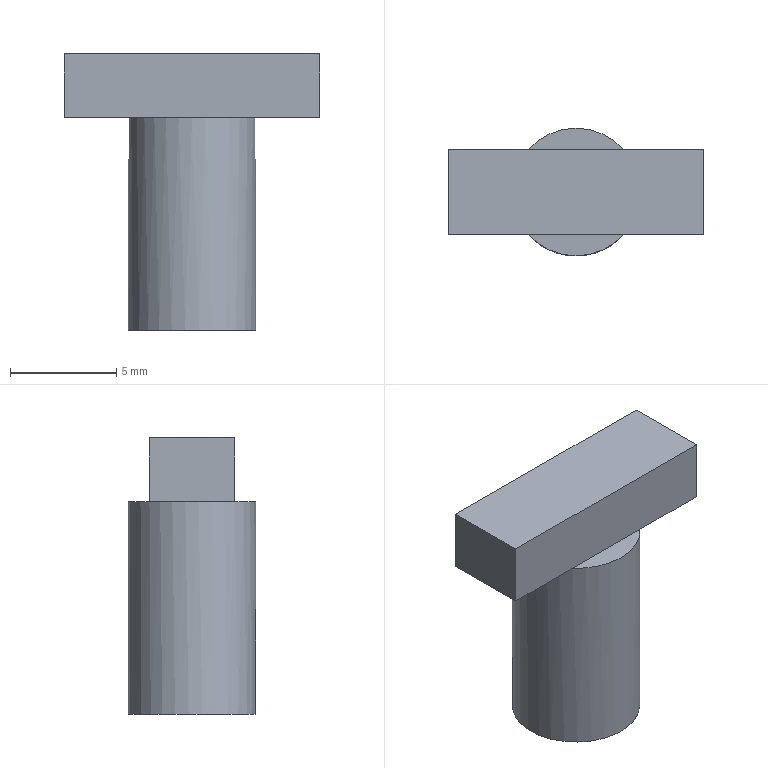Component | NX | DETENT_PIN | 1 solid | 11 faces | box 12 x 6 x 13 mm | volume 427 mm3 | plane 10 | cylinder 1 | commonest cylinder face diameters 6 x1
STEP:
#1=CARTESIAN_POINT('',(0.,0.,0.));
#2=DIRECTION('',(0.,0.,1.));
#3=DIRECTION('',(1.,0.,0.));
#4=AXIS2_PLACEMENT_3D('',#1,#2,#3);
#5=CARTESIAN_POINT('',(12.764,-2.,126.));
#6=VERTEX_POINT('',#5);
#7=CARTESIAN_POINT('',(17.236,-2.,126.));
#8=VERTEX_POINT('',#7);
#9=CARTESIAN_POINT('',(9.,-2.,126.));
#10=DIRECTION('',(1.,0.,0.));
#11=VECTOR('',#10,1.);
#12=LINE('',#9,#11);
#13=CARTESIAN_POINT('',(15.,0.,126.));
#14=DIRECTION('',(0.,0.,1.));
#15=DIRECTION('',(0.,1.,0.));
#16=AXIS2_PLACEMENT_3D('',#13,#14,#15);
#17=PLANE('',#16);
#18=CARTESIAN_POINT('',(-2.,6.));
#19=DIRECTION('',(0.,-1.));
#20=VECTOR('',#19,1.);
#21=LINE('',#18,#20);
#22=(GEOMETRIC_REPRESENTATION_CONTEXT(2)PARAMETRIC_REPRESENTATION_CONTEXT()REPRESENTATION_CONTEXT('',''));
#23=DEFINITIONAL_REPRESENTATION('',(#21),#22);
#24=PCURVE('',#17,#23);
#25=CARTESIAN_POINT('',(9.,-2.,129.));
#26=DIRECTION('',(0.,1.,0.));
#27=DIRECTION('',(0.,0.,-1.));
#28=AXIS2_PLACEMENT_3D('',#25,#26,#27);
#29=PLANE('',#28);
#30=CARTESIAN_POINT('',(3.,0.));
#31=DIRECTION('',(0.,-1.));
#32=VECTOR('',#31,1.);
#33=LINE('',#30,#32);
#34=(GEOMETRIC_REPRESENTATION_CONTEXT(2)PARAMETRIC_REPRESENTATION_CONTEXT()REPRESENTATION_CONTEXT('',''));
#35=DEFINITIONAL_REPRESENTATION('',(#33),#34);
#36=PCURVE('',#29,#35);
#37=SURFACE_CURVE('',#12,(#24,#36),.PCURVE_S1.);
#38=EDGE_CURVE('',#6,#8,#37,.T.);
#39=ORIENTED_EDGE('',*,*,#38,.F.);
#40=CARTESIAN_POINT('',(15.,0.,126.));
#41=DIRECTION('',(0.,0.,-1.));
#42=DIRECTION('',(0.,1.,0.));
#43=AXIS2_PLACEMENT_3D('',#40,#41,#42);
#44=CIRCLE('',#43,3.);
#45=CARTESIAN_POINT('',(3.,0.));
#46=CARTESIAN_POINT('',(3.,-5.196));
#47=CARTESIAN_POINT('',(-1.5,-2.598));
#48=CARTESIAN_POINT('',(-6.,-0.));
#49=CARTESIAN_POINT('',(-1.5,2.598));
#50=CARTESIAN_POINT('',(3.,5.196));
#51=CARTESIAN_POINT('',(3.,0.));
#52=(BOUNDED_CURVE()B_SPLINE_CURVE(2,(#45,#46,#47,#48,#49,#50,#51),.UNSPECIFIED.,.T.,.F.)B_SPLINE_CURVE_WITH_KNOTS((1,2,2,2,2,1),(-2.094,0.,2.094,4.189,6.283,8.378),.UNSPECIFIED.)CURVE()GEOMETRIC_REPRESENTATION_ITEM()RATIONAL_B_SPLINE_CURVE((1.,0.5,1.,0.5,1.,0.5,1.))REPRESENTATION_ITEM(''));
#53=(GEOMETRIC_REPRESENTATION_CONTEXT(2)PARAMETRIC_REPRESENTATION_CONTEXT()REPRESENTATION_CONTEXT('',''));
#54=DEFINITIONAL_REPRESENTATION('',(#52),#53);
#55=PCURVE('',#17,#54);
#56=CARTESIAN_POINT('',(15.,0.,126.));
#57=DIRECTION('',(0.,0.,-1.));
#58=DIRECTION('',(0.,1.,0.));
#59=AXIS2_PLACEMENT_3D('',#56,#57,#58);
#60=CYLINDRICAL_SURFACE('',#59,3.);
#61=CARTESIAN_POINT('',(0.,0.));
#62=DIRECTION('',(1.,0.));
#63=VECTOR('',#62,1.);
#64=LINE('',#61,#63);
#65=(GEOMETRIC_REPRESENTATION_CONTEXT(2)PARAMETRIC_REPRESENTATION_CONTEXT()REPRESENTATION_CONTEXT('',''));
#66=DEFINITIONAL_REPRESENTATION('',(#64),#65);
#67=PCURVE('',#60,#66);
#68=SURFACE_CURVE('',#44,(#55,#67),.PCURVE_S1.);
#69=EDGE_CURVE('',#8,#6,#68,.T.);
#70=ORIENTED_EDGE('',*,*,#69,.F.);
#71=EDGE_LOOP('',(#39,#70));
#72=FACE_BOUND('',#71,.T.);
#73=ADVANCED_FACE('',(#72),#17,.T.);
#74=CARTESIAN_POINT('',(15.,3.,116.));
#75=VERTEX_POINT('',#74);
#76=CARTESIAN_POINT('',(15.,0.,116.));
#77=DIRECTION('',(0.,0.,1.));
#78=DIRECTION('',(0.,1.,0.));
#79=AXIS2_PLACEMENT_3D('',#76,#77,#78);
#80=CIRCLE('',#79,3.);
#81=CARTESIAN_POINT('',(15.,0.,116.));
#82=DIRECTION('',(0.,0.,-1.));
#83=DIRECTION('',(0.,-1.,0.));
#84=AXIS2_PLACEMENT_3D('',#81,#82,#83);
#85=PLANE('',#84);
#86=CARTESIAN_POINT('',(-3.,0.));
#87=CARTESIAN_POINT('',(-3.,5.196));
#88=CARTESIAN_POINT('',(1.5,2.598));
#89=CARTESIAN_POINT('',(6.,0.));
#90=CARTESIAN_POINT('',(1.5,-2.598));
#91=CARTESIAN_POINT('',(-3.,-5.196));
#92=CARTESIAN_POINT('',(-3.,0.));
#93=(BOUNDED_CURVE()B_SPLINE_CURVE(2,(#86,#87,#88,#89,#90,#91,#92),.UNSPECIFIED.,.T.,.F.)B_SPLINE_CURVE_WITH_KNOTS((1,2,2,2,2,1),(-2.094,0.,2.094,4.189,6.283,8.378),.UNSPECIFIED.)CURVE()GEOMETRIC_REPRESENTATION_ITEM()RATIONAL_B_SPLINE_CURVE((1.,0.5,1.,0.5,1.,0.5,1.))REPRESENTATION_ITEM(''));
#94=(GEOMETRIC_REPRESENTATION_CONTEXT(2)PARAMETRIC_REPRESENTATION_CONTEXT()REPRESENTATION_CONTEXT('',''));
#95=DEFINITIONAL_REPRESENTATION('',(#93),#94);
#96=PCURVE('',#85,#95);
#97=CARTESIAN_POINT('',(6.283,10.));
#98=DIRECTION('',(-1.,0.));
#99=VECTOR('',#98,1.);
#100=LINE('',#97,#99);
#101=(GEOMETRIC_REPRESENTATION_CONTEXT(2)PARAMETRIC_REPRESENTATION_CONTEXT()REPRESENTATION_CONTEXT('',''));
#102=DEFINITIONAL_REPRESENTATION('',(#100),#101);
#103=PCURVE('',#60,#102);
#104=SURFACE_CURVE('',#80,(#96,#103),.PCURVE_S1.);
#105=EDGE_CURVE('',#75,#75,#104,.T.);
#106=ORIENTED_EDGE('',*,*,#105,.F.);
#107=EDGE_LOOP('',(#106));
#108=FACE_BOUND('',#107,.T.);
#109=ADVANCED_FACE('',(#108),#85,.T.);
#110=CARTESIAN_POINT('',(17.236,2.,126.));
#111=VERTEX_POINT('',#110);
#112=CARTESIAN_POINT('',(12.764,2.,126.));
#113=VERTEX_POINT('',#112);
#114=CARTESIAN_POINT('',(21.,2.,126.));
#115=DIRECTION('',(-1.,0.,0.));
#116=VECTOR('',#115,1.);
#117=LINE('',#114,#116);
#118=CARTESIAN_POINT('',(15.,0.,126.));
#119=DIRECTION('',(0.,0.,1.));
#120=DIRECTION('',(0.,1.,0.));
#121=AXIS2_PLACEMENT_3D('',#118,#119,#120);
#122=PLANE('',#121);
#123=CARTESIAN_POINT('',(2.,-6.));
#124=DIRECTION('',(0.,1.));
#125=VECTOR('',#124,1.);
#126=LINE('',#123,#125);
#127=(GEOMETRIC_REPRESENTATION_CONTEXT(2)PARAMETRIC_REPRESENTATION_CONTEXT()REPRESENTATION_CONTEXT('',''));
#128=DEFINITIONAL_REPRESENTATION('',(#126),#127);
#129=PCURVE('',#122,#128);
#130=CARTESIAN_POINT('',(21.,2.,129.));
#131=DIRECTION('',(0.,-1.,0.));
#132=DIRECTION('',(0.,0.,1.));
#133=AXIS2_PLACEMENT_3D('',#130,#131,#132);
#134=PLANE('',#133);
#135=CARTESIAN_POINT('',(-3.,0.));
#136=DIRECTION('',(0.,1.));
#137=VECTOR('',#136,1.);
#138=LINE('',#135,#137);
#139=(GEOMETRIC_REPRESENTATION_CONTEXT(2)PARAMETRIC_REPRESENTATION_CONTEXT()REPRESENTATION_CONTEXT('',''));
#140=DEFINITIONAL_REPRESENTATION('',(#138),#139);
#141=PCURVE('',#134,#140);
#142=SURFACE_CURVE('',#117,(#129,#141),.PCURVE_S1.);
#143=EDGE_CURVE('',#111,#113,#142,.T.);
#144=ORIENTED_EDGE('',*,*,#143,.F.);
#145=CARTESIAN_POINT('',(15.,3.,126.));
#146=VERTEX_POINT('',#145);
#147=CARTESIAN_POINT('',(15.,0.,126.));
#148=DIRECTION('',(0.,0.,-1.));
#149=DIRECTION('',(0.,1.,0.));
#150=AXIS2_PLACEMENT_3D('',#147,#148,#149);
#151=CIRCLE('',#150,3.);
#152=CARTESIAN_POINT('',(3.,0.));
#153=CARTESIAN_POINT('',(3.,-5.196));
#154=CARTESIAN_POINT('',(-1.5,-2.598));
#155=CARTESIAN_POINT('',(-6.,-0.));
#156=CARTESIAN_POINT('',(-1.5,2.598));
#157=CARTESIAN_POINT('',(3.,5.196));
#158=CARTESIAN_POINT('',(3.,0.));
#159=(BOUNDED_CURVE()B_SPLINE_CURVE(2,(#152,#153,#154,#155,#156,#157,#158),.UNSPECIFIED.,.T.,.F.)B_SPLINE_CURVE_WITH_KNOTS((1,2,2,2,2,1),(-2.094,0.,2.094,4.189,6.283,8.378),.UNSPECIFIED.)CURVE()GEOMETRIC_REPRESENTATION_ITEM()RATIONAL_B_SPLINE_CURVE((1.,0.5,1.,0.5,1.,0.5,1.))REPRESENTATION_ITEM(''));
#160=(GEOMETRIC_REPRESENTATION_CONTEXT(2)PARAMETRIC_REPRESENTATION_CONTEXT()REPRESENTATION_CONTEXT('',''));
#161=DEFINITIONAL_REPRESENTATION('',(#159),#160);
#162=PCURVE('',#122,#161);
#163=CARTESIAN_POINT('',(-6.283,0.));
#164=DIRECTION('',(1.,0.));
#165=VECTOR('',#164,1.);
#166=LINE('',#163,#165);
#167=(GEOMETRIC_REPRESENTATION_CONTEXT(2)PARAMETRIC_REPRESENTATION_CONTEXT()REPRESENTATION_CONTEXT('',''));
#168=DEFINITIONAL_REPRESENTATION('',(#166),#167);
#169=PCURVE('',#60,#168);
#170=SURFACE_CURVE('',#151,(#162,#169),.PCURVE_S1.);
#171=EDGE_CURVE('',#146,#111,#170,.T.);
#172=ORIENTED_EDGE('',*,*,#171,.F.);
#173=CARTESIAN_POINT('',(15.,0.,126.));
#174=DIRECTION('',(0.,0.,-1.));
#175=DIRECTION('',(0.,1.,0.));
#176=AXIS2_PLACEMENT_3D('',#173,#174,#175);
#177=CIRCLE('',#176,3.);
#178=CARTESIAN_POINT('',(3.,0.));
#179=CARTESIAN_POINT('',(3.,-5.196));
#180=CARTESIAN_POINT('',(-1.5,-2.598));
#181=CARTESIAN_POINT('',(-6.,-0.));
#182=CARTESIAN_POINT('',(-1.5,2.598));
#183=CARTESIAN_POINT('',(3.,5.196));
#184=CARTESIAN_POINT('',(3.,0.));
#185=(BOUNDED_CURVE()B_SPLINE_CURVE(2,(#178,#179,#180,#181,#182,#183,#184),.UNSPECIFIED.,.T.,.F.)B_SPLINE_CURVE_WITH_KNOTS((1,2,2,2,2,1),(-2.094,0.,2.094,4.189,6.283,8.378),.UNSPECIFIED.)CURVE()GEOMETRIC_REPRESENTATION_ITEM()RATIONAL_B_SPLINE_CURVE((1.,0.5,1.,0.5,1.,0.5,1.))REPRESENTATION_ITEM(''));
#186=(GEOMETRIC_REPRESENTATION_CONTEXT(2)PARAMETRIC_REPRESENTATION_CONTEXT()REPRESENTATION_CONTEXT('',''));
#187=DEFINITIONAL_REPRESENTATION('',(#185),#186);
#188=PCURVE('',#122,#187);
#189=CARTESIAN_POINT('',(0.,0.));
#190=DIRECTION('',(1.,0.));
#191=VECTOR('',#190,1.);
#192=LINE('',#189,#191);
#193=(GEOMETRIC_REPRESENTATION_CONTEXT(2)PARAMETRIC_REPRESENTATION_CONTEXT()REPRESENTATION_CONTEXT('',''));
#194=DEFINITIONAL_REPRESENTATION('',(#192),#193);
#195=PCURVE('',#60,#194);
#196=SURFACE_CURVE('',#177,(#188,#195),.PCURVE_S1.);
#197=EDGE_CURVE('',#113,#146,#196,.T.);
#198=ORIENTED_EDGE('',*,*,#197,.F.);
#199=EDGE_LOOP('',(#144,#172,#198));
#200=FACE_BOUND('',#199,.T.);
#201=ADVANCED_FACE('',(#200),#122,.T.);
#202=ORIENTED_EDGE('',*,*,#105,.T.);
#203=CARTESIAN_POINT('',(15.,3.,126.));
#204=CARTESIAN_POINT('',(15.,3.,116.));
#205=B_SPLINE_CURVE_WITH_KNOTS('',1,(#203,#204),.UNSPECIFIED.,.F.,.F.,(2,2),(0.,10.),.PIECEWISE_BEZIER_KNOTS.);
#206=CARTESIAN_POINT('',(0.,0.));
#207=DIRECTION('',(0.,1.));
#208=VECTOR('',#207,1.);
#209=LINE('',#206,#208);
#210=(GEOMETRIC_REPRESENTATION_CONTEXT(2)PARAMETRIC_REPRESENTATION_CONTEXT()REPRESENTATION_CONTEXT('',''));
#211=DEFINITIONAL_REPRESENTATION('',(#209),#210);
#212=PCURVE('',#60,#211);
#213=CARTESIAN_POINT('',(6.283,0.));
#214=DIRECTION('',(0.,1.));
#215=VECTOR('',#214,1.);
#216=LINE('',#213,#215);
#217=(GEOMETRIC_REPRESENTATION_CONTEXT(2)PARAMETRIC_REPRESENTATION_CONTEXT()REPRESENTATION_CONTEXT('',''));
#218=DEFINITIONAL_REPRESENTATION('',(#216),#217);
#219=PCURVE('',#60,#218);
#220=SEAM_CURVE('',#205,(#212,#219),.PCURVE_S1.);
#221=EDGE_CURVE('',#146,#75,#220,.T.);
#222=ORIENTED_EDGE('',*,*,#221,.F.);
#223=ORIENTED_EDGE('',*,*,#171,.T.);
#224=CARTESIAN_POINT('',(15.,0.,126.));
#225=DIRECTION('',(0.,0.,-1.));
#226=DIRECTION('',(0.,1.,0.));
#227=AXIS2_PLACEMENT_3D('',#224,#225,#226);
#228=CIRCLE('',#227,3.);
#229=CARTESIAN_POINT('',(0.,0.));
#230=DIRECTION('',(1.,0.));
#231=VECTOR('',#230,1.);
#232=LINE('',#229,#231);
#233=(GEOMETRIC_REPRESENTATION_CONTEXT(2)PARAMETRIC_REPRESENTATION_CONTEXT()REPRESENTATION_CONTEXT('',''));
#234=DEFINITIONAL_REPRESENTATION('',(#232),#233);
#235=PCURVE('',#60,#234);
#236=CARTESIAN_POINT('',(15.,0.,126.));
#237=DIRECTION('',(0.,0.,1.));
#238=DIRECTION('',(0.,1.,0.));
#239=AXIS2_PLACEMENT_3D('',#236,#237,#238);
#240=PLANE('',#239);
#241=CARTESIAN_POINT('',(3.,0.));
#242=CARTESIAN_POINT('',(3.,-5.196));
#243=CARTESIAN_POINT('',(-1.5,-2.598));
#244=CARTESIAN_POINT('',(-6.,-0.));
#245=CARTESIAN_POINT('',(-1.5,2.598));
#246=CARTESIAN_POINT('',(3.,5.196));
#247=CARTESIAN_POINT('',(3.,0.));
#248=(BOUNDED_CURVE()B_SPLINE_CURVE(2,(#241,#242,#243,#244,#245,#246,#247),.UNSPECIFIED.,.T.,.F.)B_SPLINE_CURVE_WITH_KNOTS((1,2,2,2,2,1),(-2.094,0.,2.094,4.189,6.283,8.378),.UNSPECIFIED.)CURVE()GEOMETRIC_REPRESENTATION_ITEM()RATIONAL_B_SPLINE_CURVE((1.,0.5,1.,0.5,1.,0.5,1.))REPRESENTATION_ITEM(''));
#249=(GEOMETRIC_REPRESENTATION_CONTEXT(2)PARAMETRIC_REPRESENTATION_CONTEXT()REPRESENTATION_CONTEXT('',''));
#250=DEFINITIONAL_REPRESENTATION('',(#248),#249);
#251=PCURVE('',#240,#250);
#252=SURFACE_CURVE('',#228,(#235,#251),.PCURVE_S1.);
#253=EDGE_CURVE('',#111,#8,#252,.T.);
#254=ORIENTED_EDGE('',*,*,#253,.T.);
#255=ORIENTED_EDGE('',*,*,#69,.T.);
#256=CARTESIAN_POINT('',(15.,0.,126.));
#257=DIRECTION('',(0.,0.,-1.));
#258=DIRECTION('',(0.,1.,0.));
#259=AXIS2_PLACEMENT_3D('',#256,#257,#258);
#260=CIRCLE('',#259,3.);
#261=CARTESIAN_POINT('',(0.,0.));
#262=DIRECTION('',(1.,0.));
#263=VECTOR('',#262,1.);
#264=LINE('',#261,#263);
#265=(GEOMETRIC_REPRESENTATION_CONTEXT(2)PARAMETRIC_REPRESENTATION_CONTEXT()REPRESENTATION_CONTEXT('',''));
#266=DEFINITIONAL_REPRESENTATION('',(#264),#265);
#267=PCURVE('',#60,#266);
#268=CARTESIAN_POINT('',(15.,0.,126.));
#269=DIRECTION('',(0.,0.,1.));
#270=DIRECTION('',(0.,1.,0.));
#271=AXIS2_PLACEMENT_3D('',#268,#269,#270);
#272=PLANE('',#271);
#273=CARTESIAN_POINT('',(3.,0.));
#274=CARTESIAN_POINT('',(3.,-5.196));
#275=CARTESIAN_POINT('',(-1.5,-2.598));
#276=CARTESIAN_POINT('',(-6.,-0.));
#277=CARTESIAN_POINT('',(-1.5,2.598));
#278=CARTESIAN_POINT('',(3.,5.196));
#279=CARTESIAN_POINT('',(3.,0.));
#280=(BOUNDED_CURVE()B_SPLINE_CURVE(2,(#273,#274,#275,#276,#277,#278,#279),.UNSPECIFIED.,.T.,.F.)B_SPLINE_CURVE_WITH_KNOTS((1,2,2,2,2,1),(-2.094,0.,2.094,4.189,6.283,8.378),.UNSPECIFIED.)CURVE()GEOMETRIC_REPRESENTATION_ITEM()RATIONAL_B_SPLINE_CURVE((1.,0.5,1.,0.5,1.,0.5,1.))REPRESENTATION_ITEM(''));
#281=(GEOMETRIC_REPRESENTATION_CONTEXT(2)PARAMETRIC_REPRESENTATION_CONTEXT()REPRESENTATION_CONTEXT('',''));
#282=DEFINITIONAL_REPRESENTATION('',(#280),#281);
#283=PCURVE('',#272,#282);
#284=SURFACE_CURVE('',#260,(#267,#283),.PCURVE_S1.);
#285=EDGE_CURVE('',#6,#113,#284,.T.);
#286=ORIENTED_EDGE('',*,*,#285,.T.);
#287=ORIENTED_EDGE('',*,*,#197,.T.);
#288=ORIENTED_EDGE('',*,*,#221,.T.);
#289=EDGE_LOOP('',(#202,#222,#223,#254,#255,#286,#287,#288));
#290=FACE_BOUND('',#289,.T.);
#291=ADVANCED_FACE('',(#290),#60,.T.);
#292=ORIENTED_EDGE('',*,*,#253,.F.);
#293=CARTESIAN_POINT('',(21.,2.,126.));
#294=VERTEX_POINT('',#293);
#295=CARTESIAN_POINT('',(21.,2.,126.));
#296=DIRECTION('',(-1.,0.,0.));
#297=VECTOR('',#296,1.);
#298=LINE('',#295,#297);
#299=CARTESIAN_POINT('',(2.,-6.));
#300=DIRECTION('',(0.,1.));
#301=VECTOR('',#300,1.);
#302=LINE('',#299,#301);
#303=(GEOMETRIC_REPRESENTATION_CONTEXT(2)PARAMETRIC_REPRESENTATION_CONTEXT()REPRESENTATION_CONTEXT('',''));
#304=DEFINITIONAL_REPRESENTATION('',(#302),#303);
#305=PCURVE('',#240,#304);
#306=CARTESIAN_POINT('',(-3.,0.));
#307=DIRECTION('',(0.,1.));
#308=VECTOR('',#307,1.);
#309=LINE('',#306,#308);
#310=(GEOMETRIC_REPRESENTATION_CONTEXT(2)PARAMETRIC_REPRESENTATION_CONTEXT()REPRESENTATION_CONTEXT('',''));
#311=DEFINITIONAL_REPRESENTATION('',(#309),#310);
#312=PCURVE('',#134,#311);
#313=SURFACE_CURVE('',#298,(#305,#312),.PCURVE_S1.);
#314=EDGE_CURVE('',#294,#111,#313,.T.);
#315=ORIENTED_EDGE('',*,*,#314,.F.);
#316=CARTESIAN_POINT('',(21.,-2.,126.));
#317=VERTEX_POINT('',#316);
#318=CARTESIAN_POINT('',(21.,-2.,126.));
#319=DIRECTION('',(0.,1.,0.));
#320=VECTOR('',#319,1.);
#321=LINE('',#318,#320);
#322=CARTESIAN_POINT('',(-2.,-6.));
#323=DIRECTION('',(1.,0.));
#324=VECTOR('',#323,1.);
#325=LINE('',#322,#324);
#326=(GEOMETRIC_REPRESENTATION_CONTEXT(2)PARAMETRIC_REPRESENTATION_CONTEXT()REPRESENTATION_CONTEXT('',''));
#327=DEFINITIONAL_REPRESENTATION('',(#325),#326);
#328=PCURVE('',#240,#327);
#329=CARTESIAN_POINT('',(21.,-2.,129.));
#330=DIRECTION('',(-1.,0.,0.));
#331=DIRECTION('',(0.,0.,1.));
#332=AXIS2_PLACEMENT_3D('',#329,#330,#331);
#333=PLANE('',#332);
#334=CARTESIAN_POINT('',(-3.,0.));
#335=DIRECTION('',(0.,1.));
#336=VECTOR('',#335,1.);
#337=LINE('',#334,#336);
#338=(GEOMETRIC_REPRESENTATION_CONTEXT(2)PARAMETRIC_REPRESENTATION_CONTEXT()REPRESENTATION_CONTEXT('',''));
#339=DEFINITIONAL_REPRESENTATION('',(#337),#338);
#340=PCURVE('',#333,#339);
#341=SURFACE_CURVE('',#321,(#328,#340),.PCURVE_S1.);
#342=EDGE_CURVE('',#317,#294,#341,.T.);
#343=ORIENTED_EDGE('',*,*,#342,.F.);
#344=CARTESIAN_POINT('',(9.,-2.,126.));
#345=DIRECTION('',(1.,0.,0.));
#346=VECTOR('',#345,1.);
#347=LINE('',#344,#346);
#348=CARTESIAN_POINT('',(-2.,6.));
#349=DIRECTION('',(0.,-1.));
#350=VECTOR('',#349,1.);
#351=LINE('',#348,#350);
#352=(GEOMETRIC_REPRESENTATION_CONTEXT(2)PARAMETRIC_REPRESENTATION_CONTEXT()REPRESENTATION_CONTEXT('',''));
#353=DEFINITIONAL_REPRESENTATION('',(#351),#352);
#354=PCURVE('',#240,#353);
#355=CARTESIAN_POINT('',(3.,0.));
#356=DIRECTION('',(0.,-1.));
#357=VECTOR('',#356,1.);
#358=LINE('',#355,#357);
#359=(GEOMETRIC_REPRESENTATION_CONTEXT(2)PARAMETRIC_REPRESENTATION_CONTEXT()REPRESENTATION_CONTEXT('',''));
#360=DEFINITIONAL_REPRESENTATION('',(#358),#359);
#361=PCURVE('',#29,#360);
#362=SURFACE_CURVE('',#347,(#354,#361),.PCURVE_S1.);
#363=EDGE_CURVE('',#8,#317,#362,.T.);
#364=ORIENTED_EDGE('',*,*,#363,.F.);
#365=EDGE_LOOP('',(#292,#315,#343,#364));
#366=FACE_BOUND('',#365,.T.);
#367=ADVANCED_FACE('',(#366),#240,.F.);
#368=CARTESIAN_POINT('',(9.,-2.,126.));
#369=VERTEX_POINT('',#368);
#370=CARTESIAN_POINT('',(9.,-2.,126.));
#371=DIRECTION('',(1.,0.,0.));
#372=VECTOR('',#371,1.);
#373=LINE('',#370,#372);
#374=CARTESIAN_POINT('',(3.,0.));
#375=DIRECTION('',(0.,-1.));
#376=VECTOR('',#375,1.);
#377=LINE('',#374,#376);
#378=(GEOMETRIC_REPRESENTATION_CONTEXT(2)PARAMETRIC_REPRESENTATION_CONTEXT()REPRESENTATION_CONTEXT('',''));
#379=DEFINITIONAL_REPRESENTATION('',(#377),#378);
#380=PCURVE('',#29,#379);
#381=CARTESIAN_POINT('',(-2.,6.));
#382=DIRECTION('',(0.,-1.));
#383=VECTOR('',#382,1.);
#384=LINE('',#381,#383);
#385=(GEOMETRIC_REPRESENTATION_CONTEXT(2)PARAMETRIC_REPRESENTATION_CONTEXT()REPRESENTATION_CONTEXT('',''));
#386=DEFINITIONAL_REPRESENTATION('',(#384),#385);
#387=PCURVE('',#272,#386);
#388=SURFACE_CURVE('',#373,(#380,#387),.PCURVE_S1.);
#389=EDGE_CURVE('',#369,#6,#388,.T.);
#390=ORIENTED_EDGE('',*,*,#389,.T.);
#391=ORIENTED_EDGE('',*,*,#38,.T.);
#392=ORIENTED_EDGE('',*,*,#363,.T.);
#393=CARTESIAN_POINT('',(21.,-2.,129.));
#394=VERTEX_POINT('',#393);
#395=CARTESIAN_POINT('',(21.,-2.,129.));
#396=DIRECTION('',(0.,0.,-1.));
#397=VECTOR('',#396,1.);
#398=LINE('',#395,#397);
#399=CARTESIAN_POINT('',(0.,-12.));
#400=DIRECTION('',(1.,0.));
#401=VECTOR('',#400,1.);
#402=LINE('',#399,#401);
#403=(GEOMETRIC_REPRESENTATION_CONTEXT(2)PARAMETRIC_REPRESENTATION_CONTEXT()REPRESENTATION_CONTEXT('',''));
#404=DEFINITIONAL_REPRESENTATION('',(#402),#403);
#405=PCURVE('',#29,#404);
#406=CARTESIAN_POINT('',(0.,0.));
#407=DIRECTION('',(-1.,0.));
#408=VECTOR('',#407,1.);
#409=LINE('',#406,#408);
#410=(GEOMETRIC_REPRESENTATION_CONTEXT(2)PARAMETRIC_REPRESENTATION_CONTEXT()REPRESENTATION_CONTEXT('',''));
#411=DEFINITIONAL_REPRESENTATION('',(#409),#410);
#412=PCURVE('',#333,#411);
#413=SURFACE_CURVE('',#398,(#405,#412),.PCURVE_S1.);
#414=EDGE_CURVE('',#394,#317,#413,.T.);
#415=ORIENTED_EDGE('',*,*,#414,.F.);
#416=CARTESIAN_POINT('',(9.,-2.,129.));
#417=VERTEX_POINT('',#416);
#418=CARTESIAN_POINT('',(9.,-2.,129.));
#419=DIRECTION('',(1.,0.,0.));
#420=VECTOR('',#419,1.);
#421=LINE('',#418,#420);
#422=CARTESIAN_POINT('',(0.,0.));
#423=DIRECTION('',(0.,-1.));
#424=VECTOR('',#423,1.);
#425=LINE('',#422,#424);
#426=(GEOMETRIC_REPRESENTATION_CONTEXT(2)PARAMETRIC_REPRESENTATION_CONTEXT()REPRESENTATION_CONTEXT('',''));
#427=DEFINITIONAL_REPRESENTATION('',(#425),#426);
#428=PCURVE('',#29,#427);
#429=CARTESIAN_POINT('',(15.,0.,129.));
#430=DIRECTION('',(0.,0.,1.));
#431=DIRECTION('',(0.,1.,0.));
#432=AXIS2_PLACEMENT_3D('',#429,#430,#431);
#433=PLANE('',#432);
#434=CARTESIAN_POINT('',(-2.,6.));
#435=DIRECTION('',(0.,-1.));
#436=VECTOR('',#435,1.);
#437=LINE('',#434,#436);
#438=(GEOMETRIC_REPRESENTATION_CONTEXT(2)PARAMETRIC_REPRESENTATION_CONTEXT()REPRESENTATION_CONTEXT('',''));
#439=DEFINITIONAL_REPRESENTATION('',(#437),#438);
#440=PCURVE('',#433,#439);
#441=SURFACE_CURVE('',#421,(#428,#440),.PCURVE_S1.);
#442=EDGE_CURVE('',#417,#394,#441,.T.);
#443=ORIENTED_EDGE('',*,*,#442,.F.);
#444=CARTESIAN_POINT('',(9.,-2.,129.));
#445=DIRECTION('',(0.,0.,-1.));
#446=VECTOR('',#445,1.);
#447=LINE('',#444,#446);
#448=CARTESIAN_POINT('',(0.,0.));
#449=DIRECTION('',(1.,0.));
#450=VECTOR('',#449,1.);
#451=LINE('',#448,#450);
#452=(GEOMETRIC_REPRESENTATION_CONTEXT(2)PARAMETRIC_REPRESENTATION_CONTEXT()REPRESENTATION_CONTEXT('',''));
#453=DEFINITIONAL_REPRESENTATION('',(#451),#452);
#454=PCURVE('',#29,#453);
#455=CARTESIAN_POINT('',(9.,2.,129.));
#456=DIRECTION('',(1.,0.,0.));
#457=DIRECTION('',(0.,0.,-1.));
#458=AXIS2_PLACEMENT_3D('',#455,#456,#457);
#459=PLANE('',#458);
#460=CARTESIAN_POINT('',(0.,-4.));
#461=DIRECTION('',(1.,0.));
#462=VECTOR('',#461,1.);
#463=LINE('',#460,#462);
#464=(GEOMETRIC_REPRESENTATION_CONTEXT(2)PARAMETRIC_REPRESENTATION_CONTEXT()REPRESENTATION_CONTEXT('',''));
#465=DEFINITIONAL_REPRESENTATION('',(#463),#464);
#466=PCURVE('',#459,#465);
#467=SURFACE_CURVE('',#447,(#454,#466),.PCURVE_S1.);
#468=EDGE_CURVE('',#417,#369,#467,.T.);
#469=ORIENTED_EDGE('',*,*,#468,.T.);
#470=EDGE_LOOP('',(#390,#391,#392,#415,#443,#469));
#471=FACE_BOUND('',#470,.T.);
#472=ADVANCED_FACE('',(#471),#29,.F.);
#473=ORIENTED_EDGE('',*,*,#342,.T.);
#474=CARTESIAN_POINT('',(21.,2.,129.));
#475=VERTEX_POINT('',#474);
#476=CARTESIAN_POINT('',(21.,2.,129.));
#477=DIRECTION('',(0.,0.,-1.));
#478=VECTOR('',#477,1.);
#479=LINE('',#476,#478);
#480=CARTESIAN_POINT('',(0.,4.));
#481=DIRECTION('',(-1.,0.));
#482=VECTOR('',#481,1.);
#483=LINE('',#480,#482);
#484=(GEOMETRIC_REPRESENTATION_CONTEXT(2)PARAMETRIC_REPRESENTATION_CONTEXT()REPRESENTATION_CONTEXT('',''));
#485=DEFINITIONAL_REPRESENTATION('',(#483),#484);
#486=PCURVE('',#333,#485);
#487=CARTESIAN_POINT('',(0.,0.));
#488=DIRECTION('',(-1.,0.));
#489=VECTOR('',#488,1.);
#490=LINE('',#487,#489);
#491=(GEOMETRIC_REPRESENTATION_CONTEXT(2)PARAMETRIC_REPRESENTATION_CONTEXT()REPRESENTATION_CONTEXT('',''));
#492=DEFINITIONAL_REPRESENTATION('',(#490),#491);
#493=PCURVE('',#134,#492);
#494=SURFACE_CURVE('',#479,(#486,#493),.PCURVE_S1.);
#495=EDGE_CURVE('',#475,#294,#494,.T.);
#496=ORIENTED_EDGE('',*,*,#495,.F.);
#497=CARTESIAN_POINT('',(21.,-2.,129.));
#498=DIRECTION('',(0.,1.,0.));
#499=VECTOR('',#498,1.);
#500=LINE('',#497,#499);
#501=CARTESIAN_POINT('',(0.,0.));
#502=DIRECTION('',(0.,1.));
#503=VECTOR('',#502,1.);
#504=LINE('',#501,#503);
#505=(GEOMETRIC_REPRESENTATION_CONTEXT(2)PARAMETRIC_REPRESENTATION_CONTEXT()REPRESENTATION_CONTEXT('',''));
#506=DEFINITIONAL_REPRESENTATION('',(#504),#505);
#507=PCURVE('',#333,#506);
#508=CARTESIAN_POINT('',(-2.,-6.));
#509=DIRECTION('',(1.,0.));
#510=VECTOR('',#509,1.);
#511=LINE('',#508,#510);
#512=(GEOMETRIC_REPRESENTATION_CONTEXT(2)PARAMETRIC_REPRESENTATION_CONTEXT()REPRESENTATION_CONTEXT('',''));
#513=DEFINITIONAL_REPRESENTATION('',(#511),#512);
#514=PCURVE('',#433,#513);
#515=SURFACE_CURVE('',#500,(#507,#514),.PCURVE_S1.);
#516=EDGE_CURVE('',#394,#475,#515,.T.);
#517=ORIENTED_EDGE('',*,*,#516,.F.);
#518=ORIENTED_EDGE('',*,*,#414,.T.);
#519=EDGE_LOOP('',(#473,#496,#517,#518));
#520=FACE_BOUND('',#519,.T.);
#521=ADVANCED_FACE('',(#520),#333,.F.);
#522=ORIENTED_EDGE('',*,*,#314,.T.);
#523=ORIENTED_EDGE('',*,*,#143,.T.);
#524=CARTESIAN_POINT('',(9.,2.,126.));
#525=VERTEX_POINT('',#524);
#526=CARTESIAN_POINT('',(21.,2.,126.));
#527=DIRECTION('',(-1.,0.,0.));
#528=VECTOR('',#527,1.);
#529=LINE('',#526,#528);
#530=CARTESIAN_POINT('',(-3.,0.));
#531=DIRECTION('',(0.,1.));
#532=VECTOR('',#531,1.);
#533=LINE('',#530,#532);
#534=(GEOMETRIC_REPRESENTATION_CONTEXT(2)PARAMETRIC_REPRESENTATION_CONTEXT()REPRESENTATION_CONTEXT('',''));
#535=DEFINITIONAL_REPRESENTATION('',(#533),#534);
#536=PCURVE('',#134,#535);
#537=CARTESIAN_POINT('',(2.,-6.));
#538=DIRECTION('',(0.,1.));
#539=VECTOR('',#538,1.);
#540=LINE('',#537,#539);
#541=(GEOMETRIC_REPRESENTATION_CONTEXT(2)PARAMETRIC_REPRESENTATION_CONTEXT()REPRESENTATION_CONTEXT('',''));
#542=DEFINITIONAL_REPRESENTATION('',(#540),#541);
#543=PCURVE('',#272,#542);
#544=SURFACE_CURVE('',#529,(#536,#543),.PCURVE_S1.);
#545=EDGE_CURVE('',#113,#525,#544,.T.);
#546=ORIENTED_EDGE('',*,*,#545,.T.);
#547=CARTESIAN_POINT('',(9.,2.,129.));
#548=VERTEX_POINT('',#547);
#549=CARTESIAN_POINT('',(9.,2.,129.));
#550=DIRECTION('',(0.,0.,-1.));
#551=VECTOR('',#550,1.);
#552=LINE('',#549,#551);
#553=CARTESIAN_POINT('',(0.,12.));
#554=DIRECTION('',(-1.,0.));
#555=VECTOR('',#554,1.);
#556=LINE('',#553,#555);
#557=(GEOMETRIC_REPRESENTATION_CONTEXT(2)PARAMETRIC_REPRESENTATION_CONTEXT()REPRESENTATION_CONTEXT('',''));
#558=DEFINITIONAL_REPRESENTATION('',(#556),#557);
#559=PCURVE('',#134,#558);
#560=CARTESIAN_POINT('',(0.,0.));
#561=DIRECTION('',(1.,0.));
#562=VECTOR('',#561,1.);
#563=LINE('',#560,#562);
#564=(GEOMETRIC_REPRESENTATION_CONTEXT(2)PARAMETRIC_REPRESENTATION_CONTEXT()REPRESENTATION_CONTEXT('',''));
#565=DEFINITIONAL_REPRESENTATION('',(#563),#564);
#566=PCURVE('',#459,#565);
#567=SURFACE_CURVE('',#552,(#559,#566),.PCURVE_S1.);
#568=EDGE_CURVE('',#548,#525,#567,.T.);
#569=ORIENTED_EDGE('',*,*,#568,.F.);
#570=CARTESIAN_POINT('',(21.,2.,129.));
#571=DIRECTION('',(-1.,0.,0.));
#572=VECTOR('',#571,1.);
#573=LINE('',#570,#572);
#574=CARTESIAN_POINT('',(0.,0.));
#575=DIRECTION('',(0.,1.));
#576=VECTOR('',#575,1.);
#577=LINE('',#574,#576);
#578=(GEOMETRIC_REPRESENTATION_CONTEXT(2)PARAMETRIC_REPRESENTATION_CONTEXT()REPRESENTATION_CONTEXT('',''));
#579=DEFINITIONAL_REPRESENTATION('',(#577),#578);
#580=PCURVE('',#134,#579);
#581=CARTESIAN_POINT('',(2.,-6.));
#582=DIRECTION('',(0.,1.));
#583=VECTOR('',#582,1.);
#584=LINE('',#581,#583);
#585=(GEOMETRIC_REPRESENTATION_CONTEXT(2)PARAMETRIC_REPRESENTATION_CONTEXT()REPRESENTATION_CONTEXT('',''));
#586=DEFINITIONAL_REPRESENTATION('',(#584),#585);
#587=PCURVE('',#433,#586);
#588=SURFACE_CURVE('',#573,(#580,#587),.PCURVE_S1.);
#589=EDGE_CURVE('',#475,#548,#588,.T.);
#590=ORIENTED_EDGE('',*,*,#589,.F.);
#591=ORIENTED_EDGE('',*,*,#495,.T.);
#592=EDGE_LOOP('',(#522,#523,#546,#569,#590,#591));
#593=FACE_BOUND('',#592,.T.);
#594=ADVANCED_FACE('',(#593),#134,.F.);
#595=CARTESIAN_POINT('',(9.,2.,126.));
#596=DIRECTION('',(0.,-1.,0.));
#597=VECTOR('',#596,1.);
#598=LINE('',#595,#597);
#599=CARTESIAN_POINT('',(3.,0.));
#600=DIRECTION('',(0.,-1.));
#601=VECTOR('',#600,1.);
#602=LINE('',#599,#601);
#603=(GEOMETRIC_REPRESENTATION_CONTEXT(2)PARAMETRIC_REPRESENTATION_CONTEXT()REPRESENTATION_CONTEXT('',''));
#604=DEFINITIONAL_REPRESENTATION('',(#602),#603);
#605=PCURVE('',#459,#604);
#606=CARTESIAN_POINT('',(2.,6.));
#607=DIRECTION('',(-1.,0.));
#608=VECTOR('',#607,1.);
#609=LINE('',#606,#608);
#610=(GEOMETRIC_REPRESENTATION_CONTEXT(2)PARAMETRIC_REPRESENTATION_CONTEXT()REPRESENTATION_CONTEXT('',''));
#611=DEFINITIONAL_REPRESENTATION('',(#609),#610);
#612=PCURVE('',#272,#611);
#613=SURFACE_CURVE('',#598,(#605,#612),.PCURVE_S1.);
#614=EDGE_CURVE('',#525,#369,#613,.T.);
#615=ORIENTED_EDGE('',*,*,#614,.T.);
#616=ORIENTED_EDGE('',*,*,#468,.F.);
#617=CARTESIAN_POINT('',(9.,2.,129.));
#618=DIRECTION('',(0.,-1.,0.));
#619=VECTOR('',#618,1.);
#620=LINE('',#617,#619);
#621=CARTESIAN_POINT('',(0.,0.));
#622=DIRECTION('',(0.,-1.));
#623=VECTOR('',#622,1.);
#624=LINE('',#621,#623);
#625=(GEOMETRIC_REPRESENTATION_CONTEXT(2)PARAMETRIC_REPRESENTATION_CONTEXT()REPRESENTATION_CONTEXT('',''));
#626=DEFINITIONAL_REPRESENTATION('',(#624),#625);
#627=PCURVE('',#459,#626);
#628=CARTESIAN_POINT('',(2.,6.));
#629=DIRECTION('',(-1.,0.));
#630=VECTOR('',#629,1.);
#631=LINE('',#628,#630);
#632=(GEOMETRIC_REPRESENTATION_CONTEXT(2)PARAMETRIC_REPRESENTATION_CONTEXT()REPRESENTATION_CONTEXT('',''));
#633=DEFINITIONAL_REPRESENTATION('',(#631),#632);
#634=PCURVE('',#433,#633);
#635=SURFACE_CURVE('',#620,(#627,#634),.PCURVE_S1.);
#636=EDGE_CURVE('',#548,#417,#635,.T.);
#637=ORIENTED_EDGE('',*,*,#636,.F.);
#638=ORIENTED_EDGE('',*,*,#568,.T.);
#639=EDGE_LOOP('',(#615,#616,#637,#638));
#640=FACE_BOUND('',#639,.T.);
#641=ADVANCED_FACE('',(#640),#459,.F.);
#642=ORIENTED_EDGE('',*,*,#442,.T.);
#643=ORIENTED_EDGE('',*,*,#516,.T.);
#644=ORIENTED_EDGE('',*,*,#589,.T.);
#645=ORIENTED_EDGE('',*,*,#636,.T.);
#646=EDGE_LOOP('',(#642,#643,#644,#645));
#647=FACE_BOUND('',#646,.T.);
#648=ADVANCED_FACE('',(#647),#433,.T.);
#649=ORIENTED_EDGE('',*,*,#285,.F.);
#650=ORIENTED_EDGE('',*,*,#389,.F.);
#651=ORIENTED_EDGE('',*,*,#614,.F.);
#652=ORIENTED_EDGE('',*,*,#545,.F.);
#653=EDGE_LOOP('',(#649,#650,#651,#652));
#654=FACE_BOUND('',#653,.T.);
#655=ADVANCED_FACE('',(#654),#272,.F.);
#656=CLOSED_SHELL('',(#73,#109,#201,#291,#367,#472,#521,#594,#641,#648,#655));
#657=MANIFOLD_SOLID_BREP('',#656);
#658=(LENGTH_UNIT()NAMED_UNIT(*)SI_UNIT(.MILLI.,.METRE.));
#659=UNCERTAINTY_MEASURE_WITH_UNIT(LENGTH_MEASURE(0.000001),#658,'','');
#660=(NAMED_UNIT(*)PLANE_ANGLE_UNIT()SI_UNIT($,.RADIAN.));
#661=(NAMED_UNIT(*)SI_UNIT($,.STERADIAN.)SOLID_ANGLE_UNIT());
#662=(GEOMETRIC_REPRESENTATION_CONTEXT(3)GLOBAL_UNCERTAINTY_ASSIGNED_CONTEXT((#659))GLOBAL_UNIT_ASSIGNED_CONTEXT((#658,#660,#661))REPRESENTATION_CONTEXT('',''));
#663=ADVANCED_BREP_SHAPE_REPRESENTATION('',(#4,#657),#662);